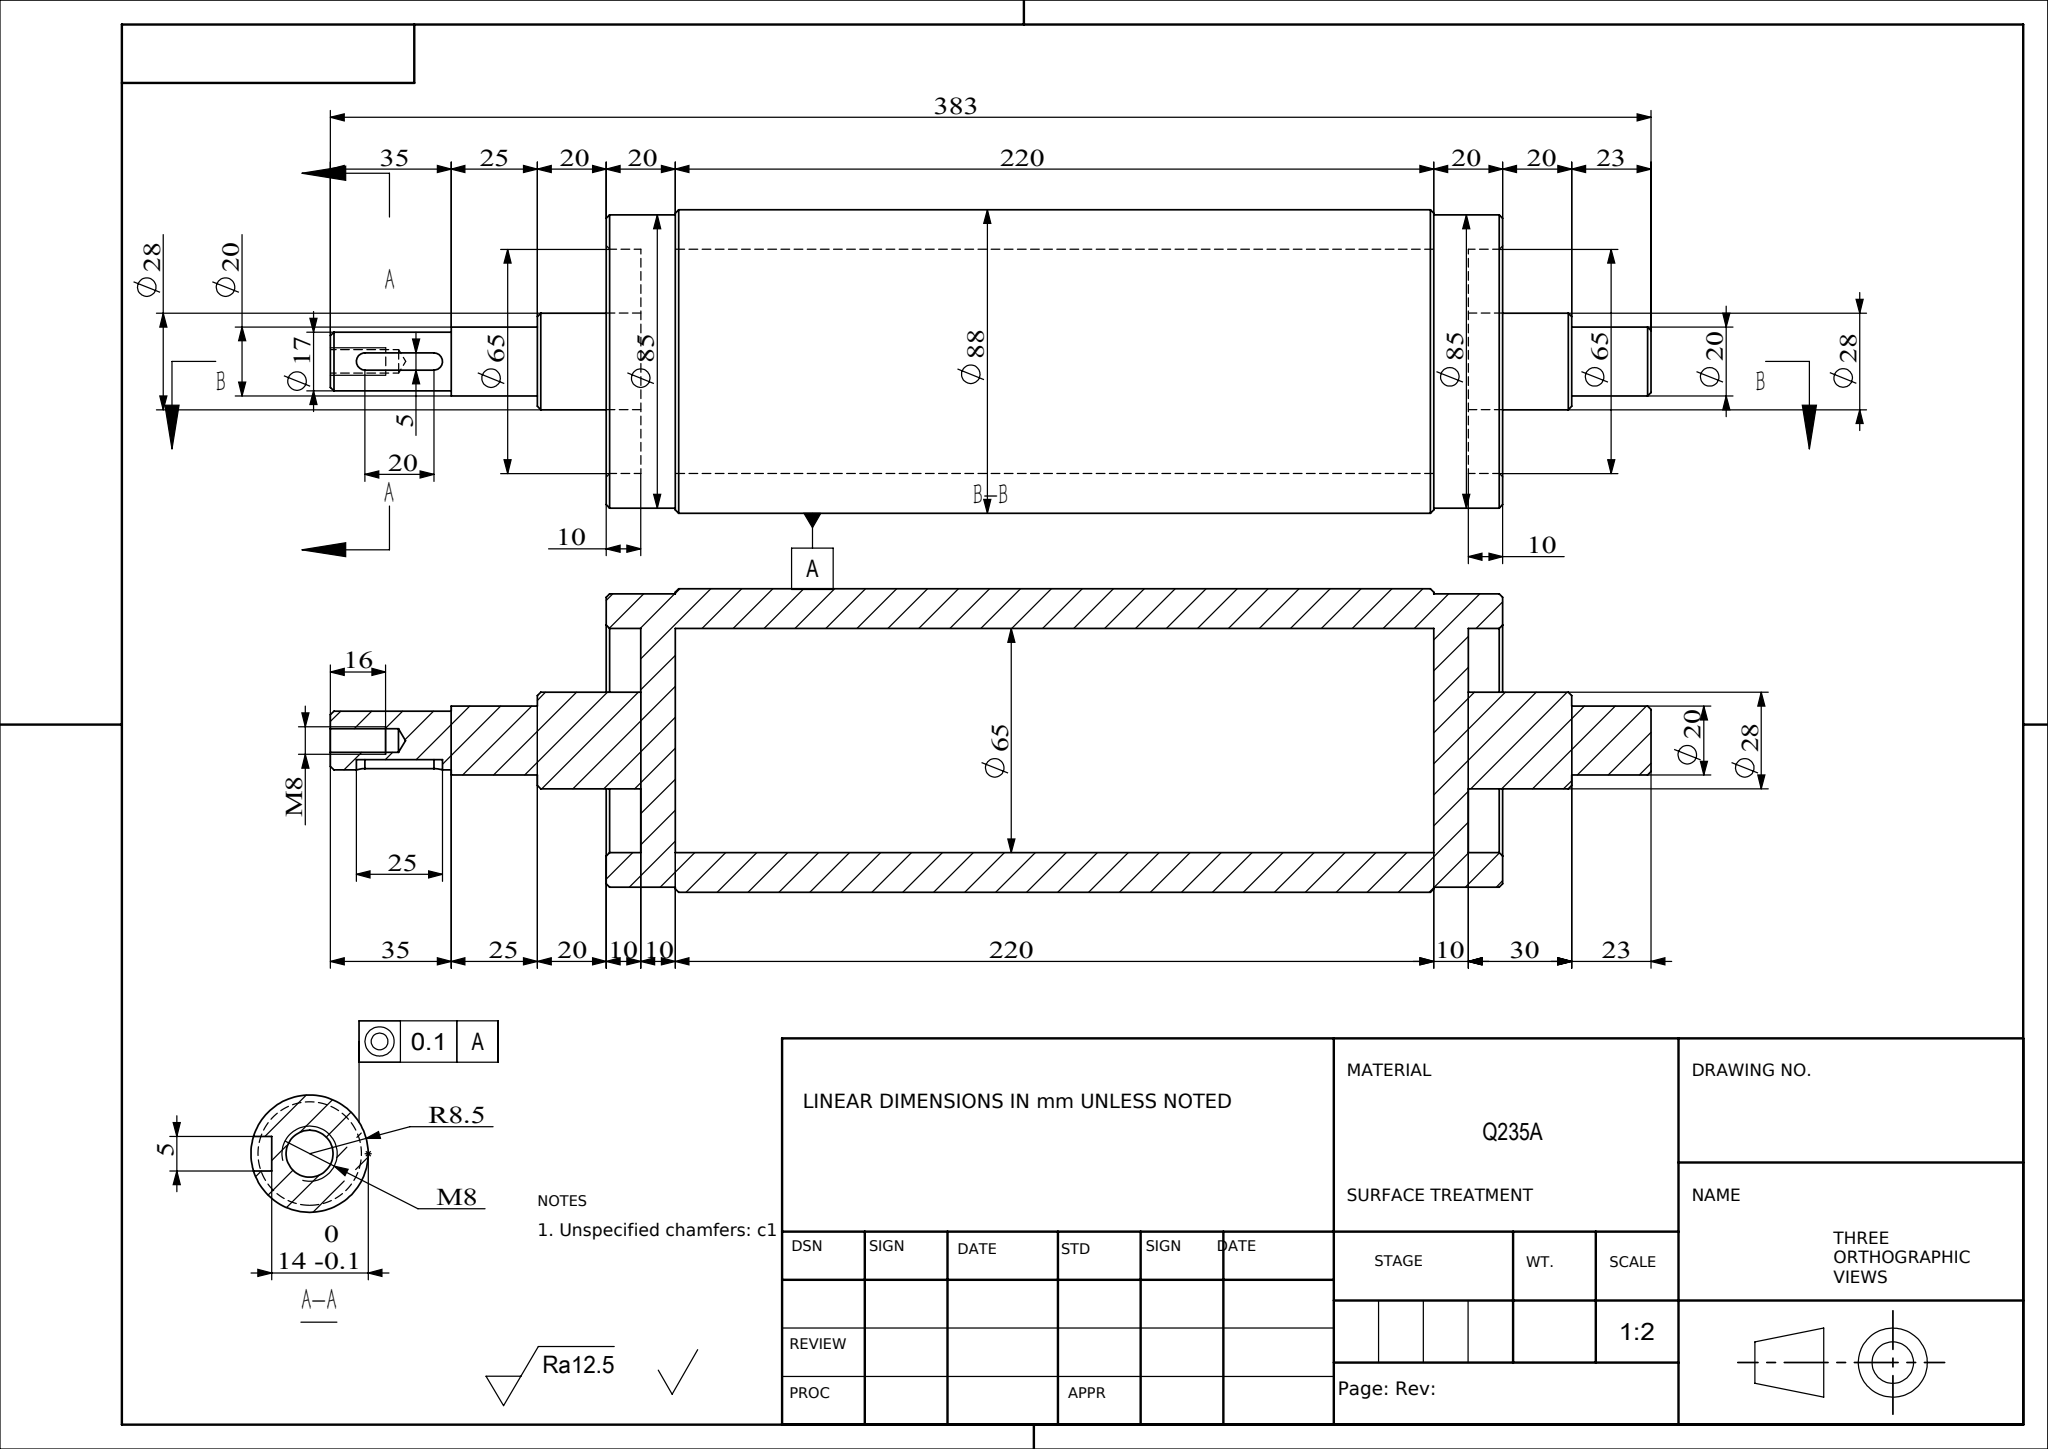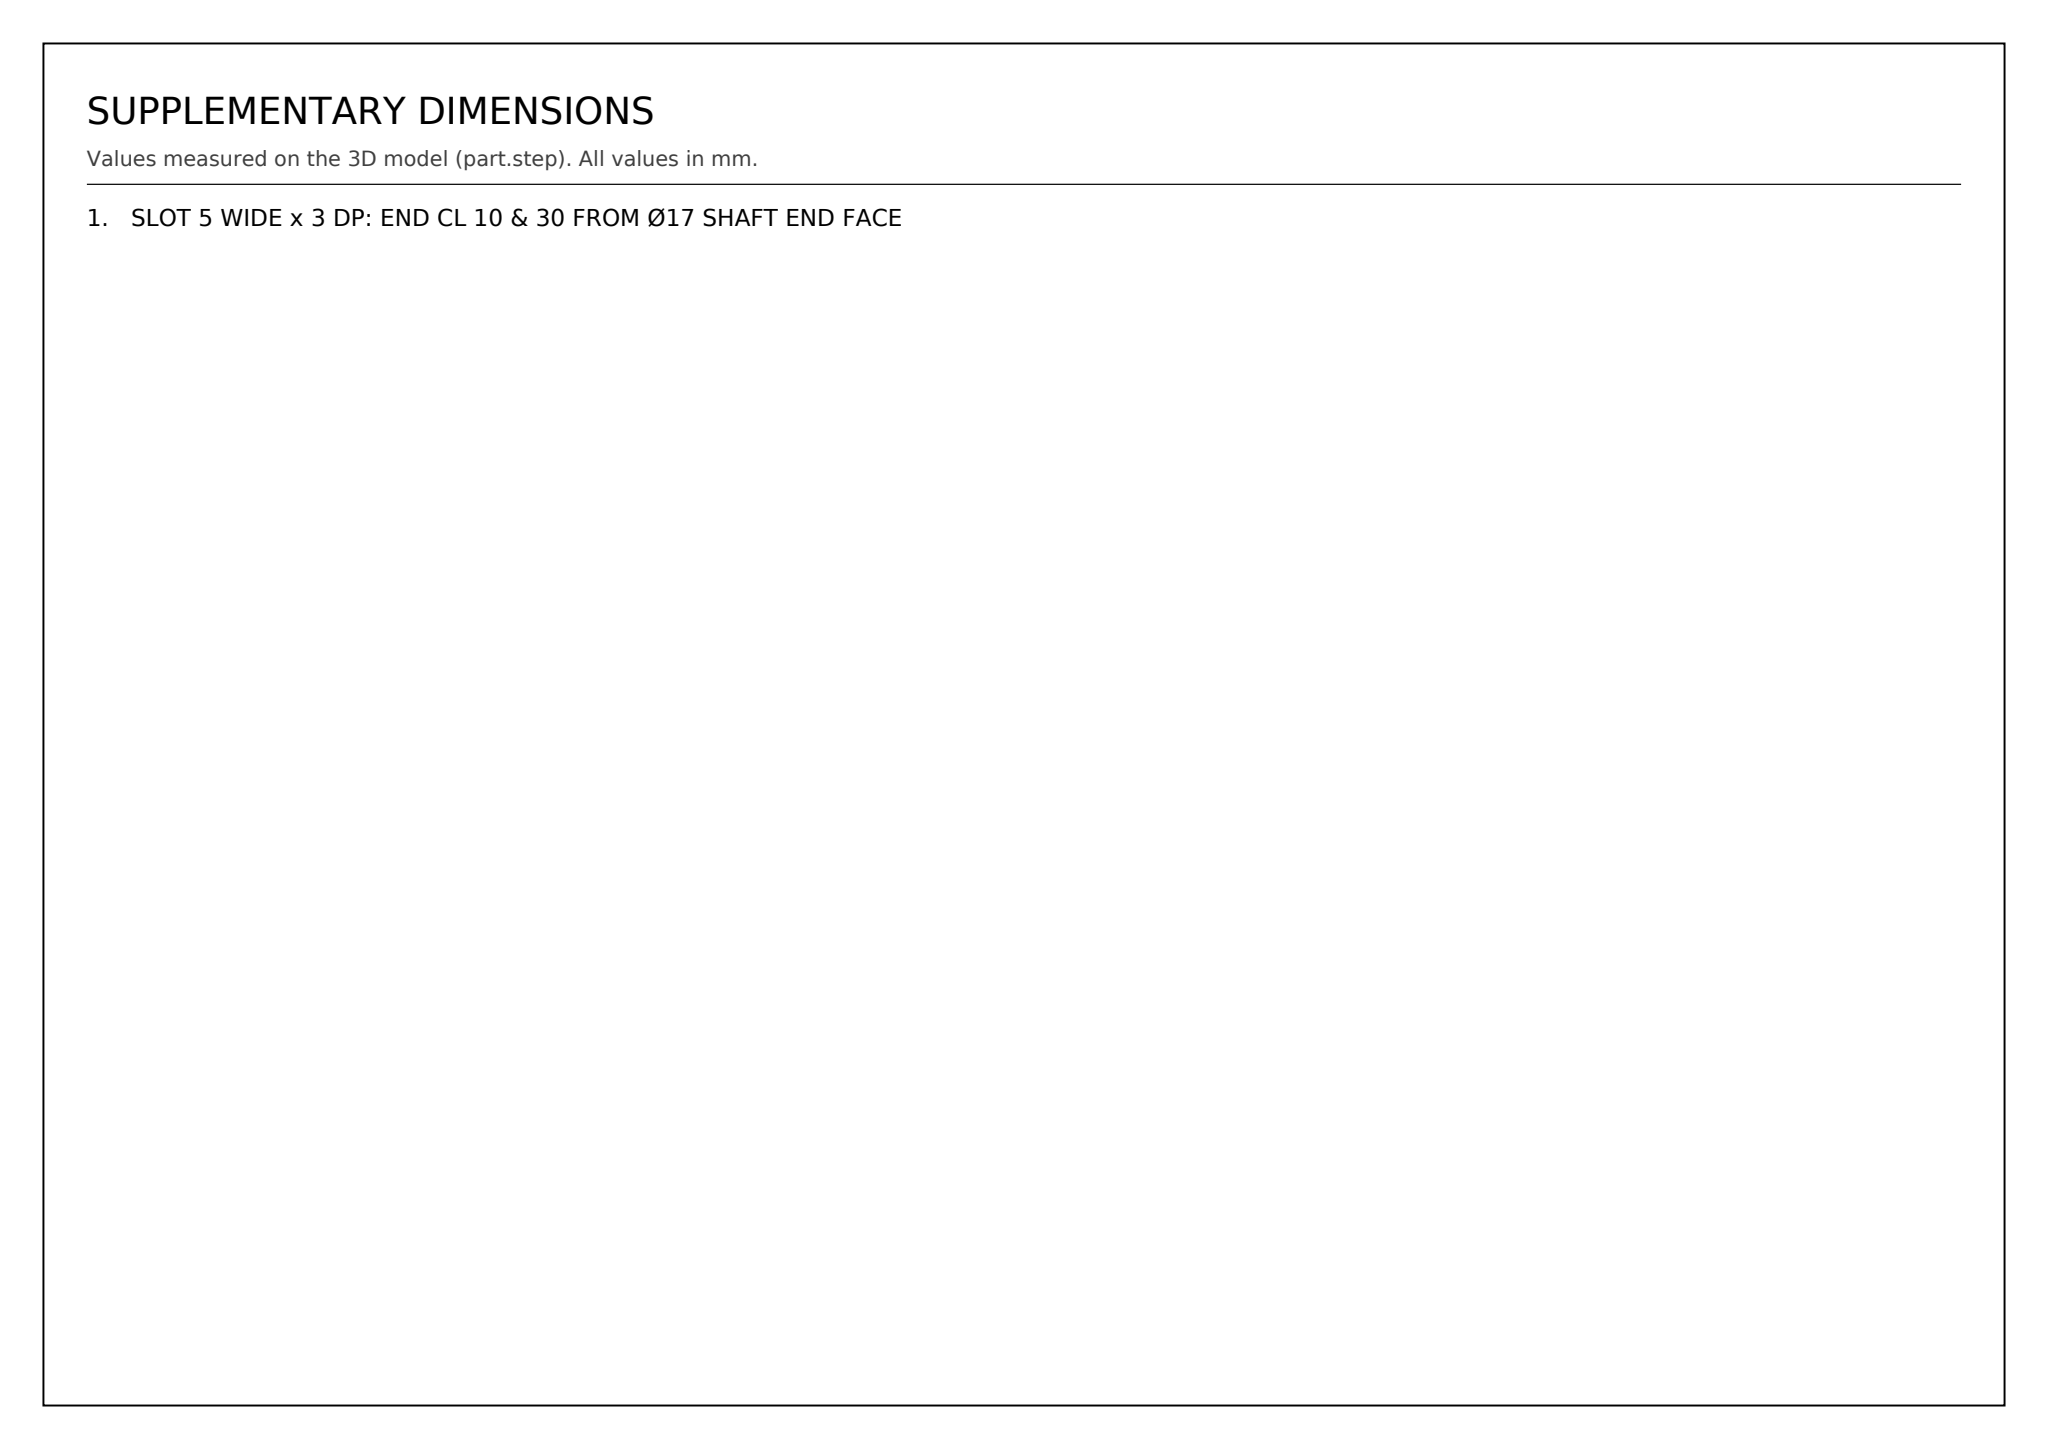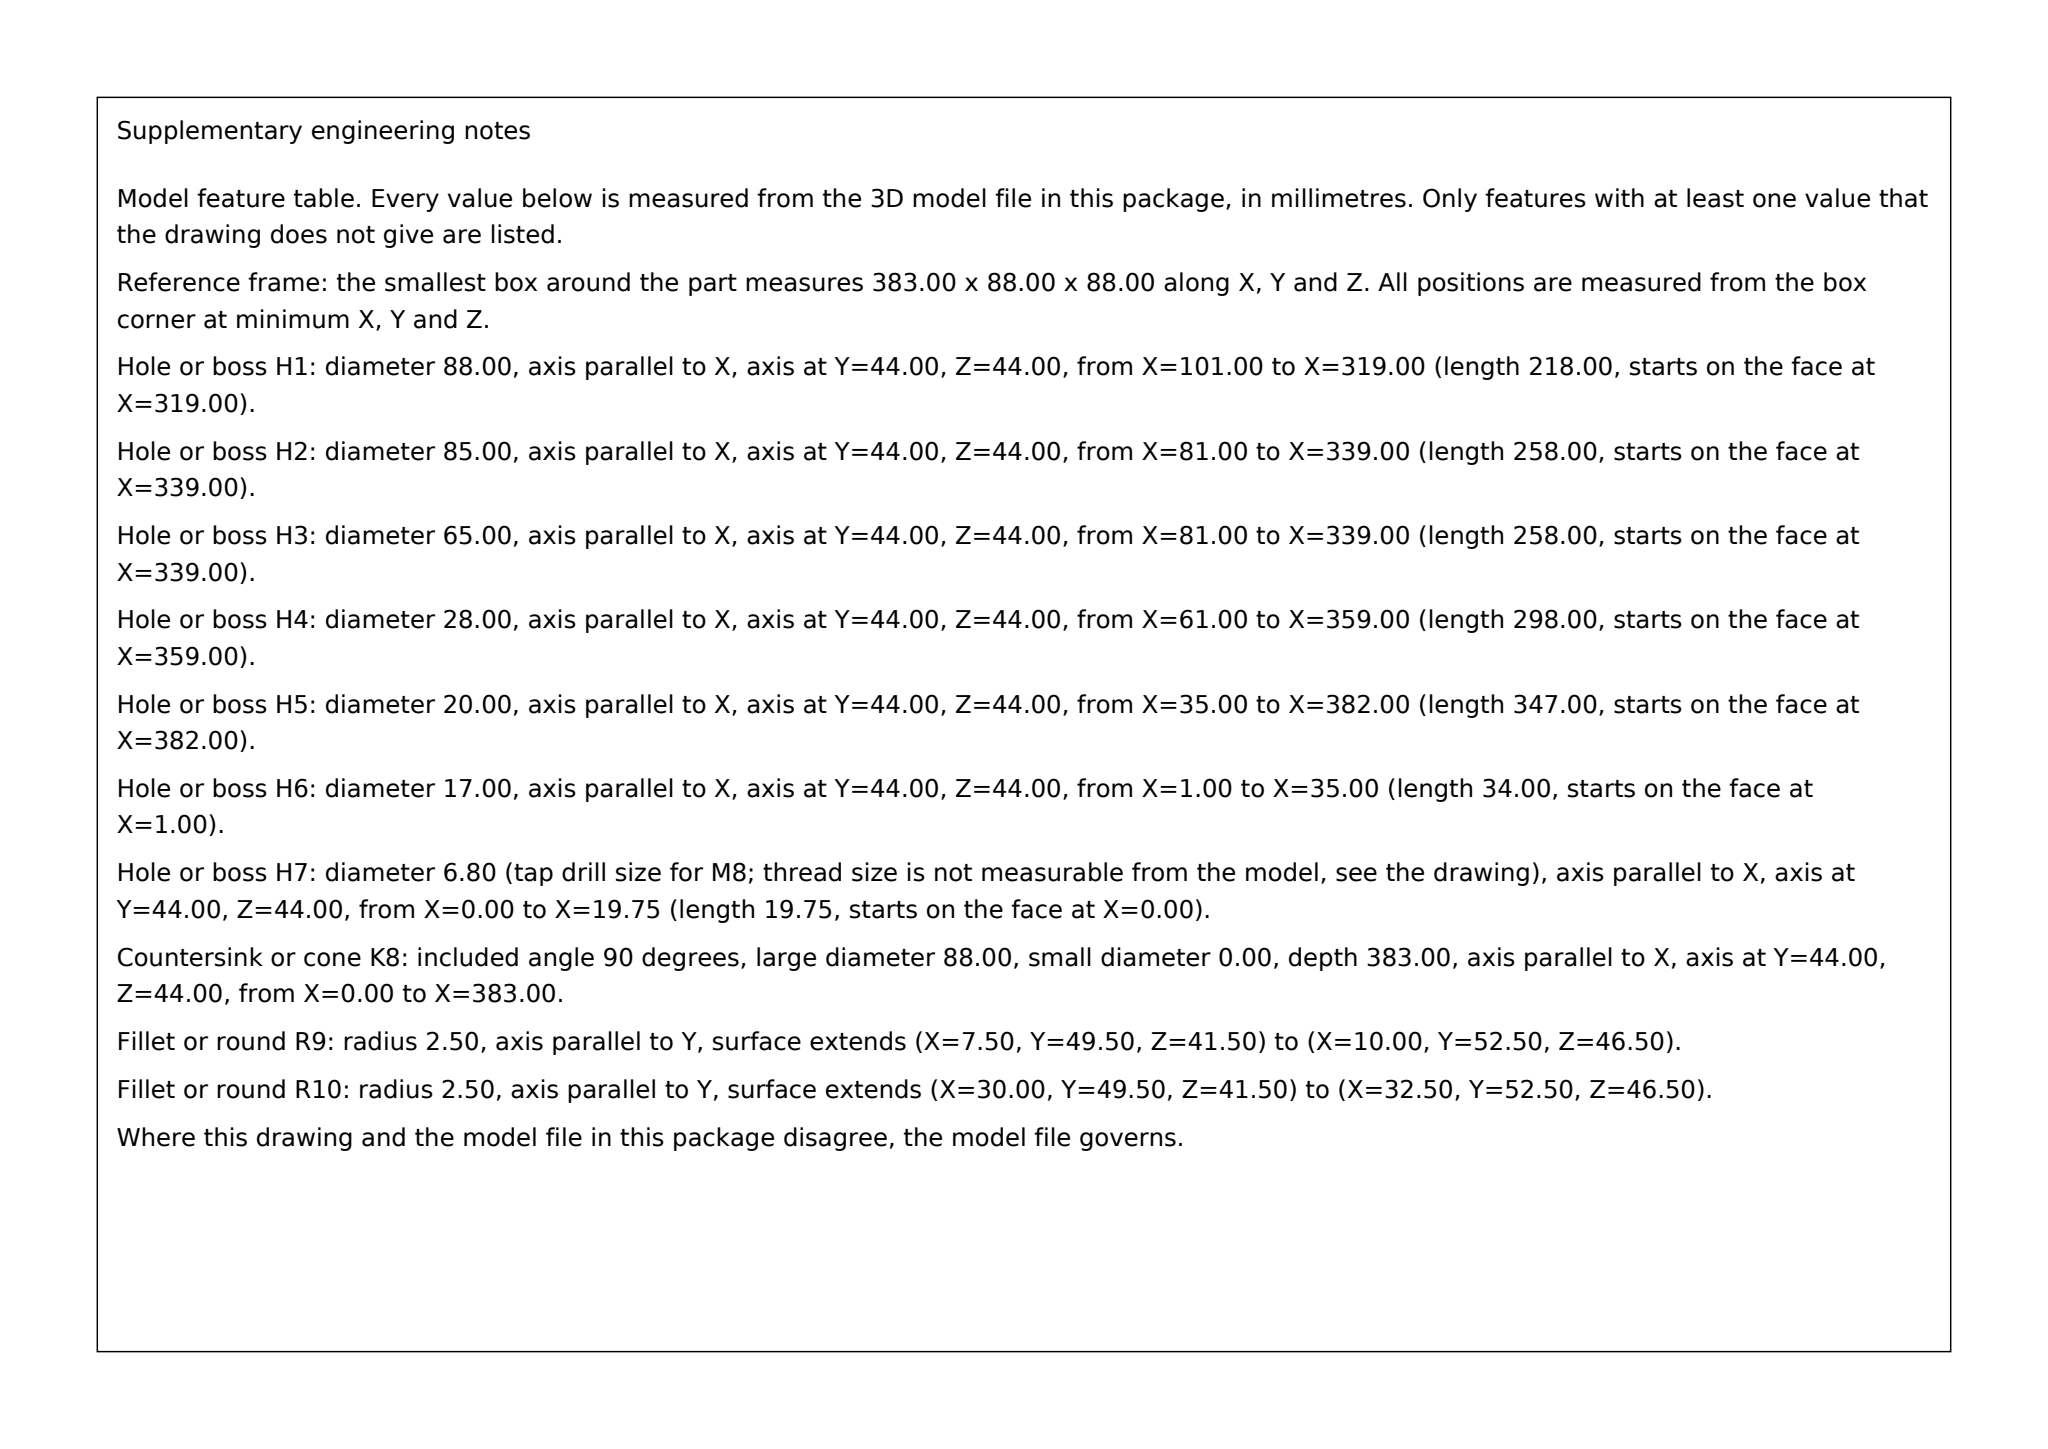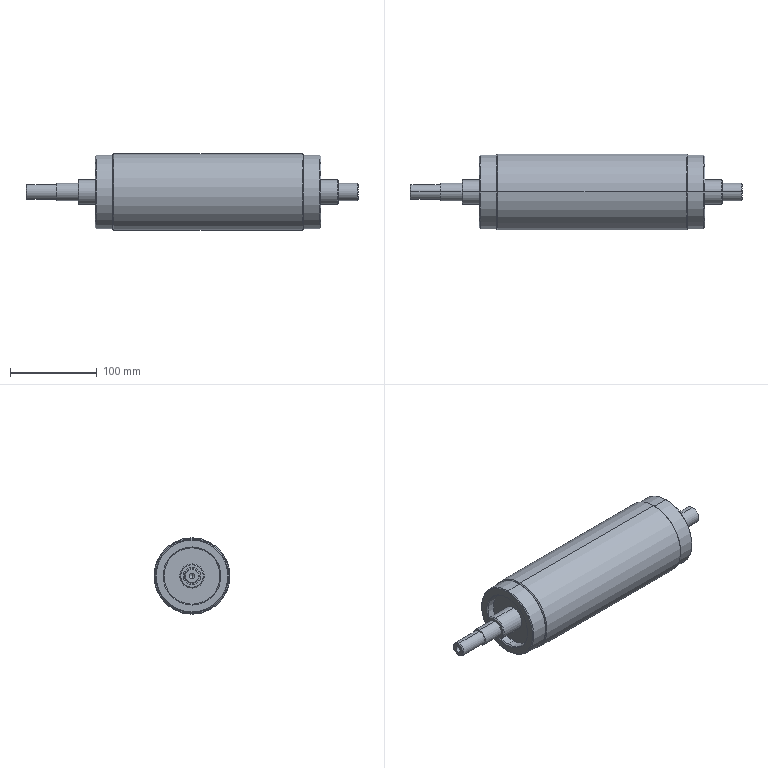Part | SolidWorks | mm | 1 solid | 64 faces | box 383 x 88 x 88 mm | volume 826648 mm3 | cylinder 26 | cone 22 | plane 16 | commonest cylinder face diameters 65 x6 85 x4 20 x4 28 x4 6.8 x2 88 x2 17 x2 5 x2
Drawing notes:
SLOT 5 WIDE x 3 DP: END CL 10 & 30 FROM Ø17 SHAFT END FACE | from the solid: Dia 5 y-axis cylinders at x=10 and x=30, len 3, from y=52.5 (Ø17) to y=49.5 plane; 20 between centres